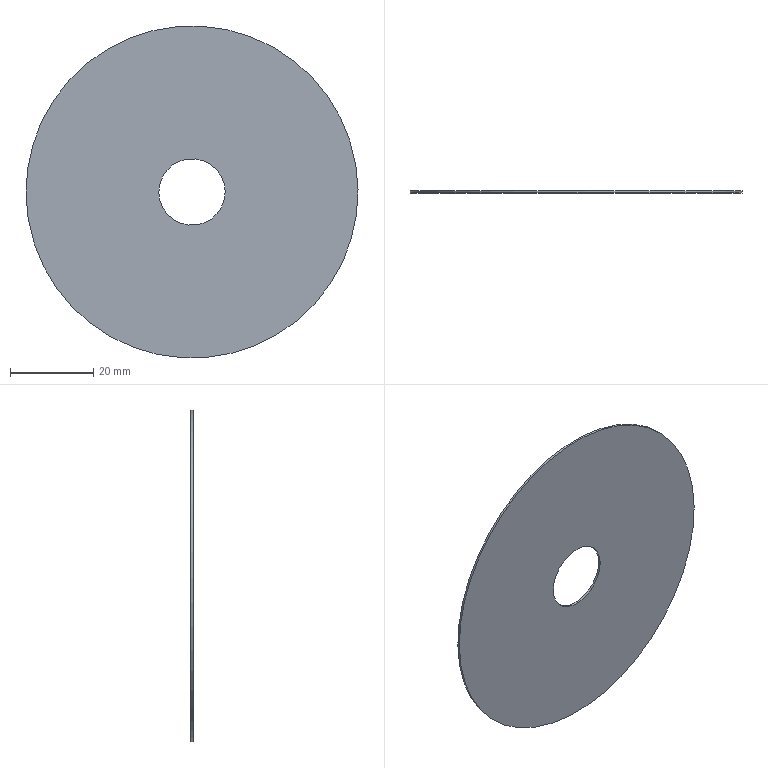Component | NX | BLADE | 1 solid | 4 faces | box 80 x 0.5 x 80 mm | volume 2413 mm3 | cylinder 2 | plane 2 | commonest cylinder face diameters 80 x1 16 x1
STEP:
#1=CARTESIAN_POINT('',(0.,0.,0.));
#2=DIRECTION('',(0.,0.,1.));
#3=DIRECTION('',(1.,0.,0.));
#4=AXIS2_PLACEMENT_3D('',#1,#2,#3);
#5=CARTESIAN_POINT('',(-471.672,8.4,378.045));
#6=VERTEX_POINT('',#5);
#7=CARTESIAN_POINT('',(-431.676,8.4,378.556));
#8=DIRECTION('',(0.,1.,0.));
#9=DIRECTION('',(-0.9999,0.,-0.01278));
#10=AXIS2_PLACEMENT_3D('',#7,#8,#9);
#11=CIRCLE('',#10,40.);
#12=CARTESIAN_POINT('',(-431.676,8.4,378.556));
#13=DIRECTION('',(0.,-1.,0.));
#14=DIRECTION('',(-0.01278,0.,0.9999));
#15=AXIS2_PLACEMENT_3D('',#12,#13,#14);
#16=CYLINDRICAL_SURFACE('',#15,40.);
#17=CARTESIAN_POINT('',(7.854,0.));
#18=DIRECTION('',(-1.,0.));
#19=VECTOR('',#18,1.);
#20=LINE('',#17,#19);
#21=(GEOMETRIC_REPRESENTATION_CONTEXT(2)PARAMETRIC_REPRESENTATION_CONTEXT()REPRESENTATION_CONTEXT('',''));
#22=DEFINITIONAL_REPRESENTATION('',(#20),#21);
#23=PCURVE('',#16,#22);
#24=CARTESIAN_POINT('',(-431.676,8.4,378.556));
#25=DIRECTION('',(0.,1.,0.));
#26=DIRECTION('',(0.01278,0.,-0.9999));
#27=AXIS2_PLACEMENT_3D('',#24,#25,#26);
#28=PLANE('',#27);
#29=CARTESIAN_POINT('',(0.,0.));
#30=DIRECTION('',(-0.,1.));
#31=AXIS2_PLACEMENT_2D('',#29,#30);
#32=CIRCLE('',#31,40.);
#33=(GEOMETRIC_REPRESENTATION_CONTEXT(2)PARAMETRIC_REPRESENTATION_CONTEXT()REPRESENTATION_CONTEXT('',''));
#34=DEFINITIONAL_REPRESENTATION('',(#32),#33);
#35=PCURVE('',#28,#34);
#36=SURFACE_CURVE('',#11,(#23,#35),.PCURVE_S1.);
#37=EDGE_CURVE('',#6,#6,#36,.T.);
#38=ORIENTED_EDGE('',*,*,#37,.F.);
#39=CARTESIAN_POINT('',(-471.672,7.9,378.045));
#40=VERTEX_POINT('',#39);
#41=CARTESIAN_POINT('',(-471.672,8.4,378.045));
#42=CARTESIAN_POINT('',(-471.672,7.9,378.045));
#43=B_SPLINE_CURVE_WITH_KNOTS('',1,(#41,#42),.UNSPECIFIED.,.F.,.F.,(2,2),(0.,0.5),.PIECEWISE_BEZIER_KNOTS.);
#44=CARTESIAN_POINT('',(7.854,0.));
#45=DIRECTION('',(0.,1.));
#46=VECTOR('',#45,1.);
#47=LINE('',#44,#46);
#48=(GEOMETRIC_REPRESENTATION_CONTEXT(2)PARAMETRIC_REPRESENTATION_CONTEXT()REPRESENTATION_CONTEXT('',''));
#49=DEFINITIONAL_REPRESENTATION('',(#47),#48);
#50=PCURVE('',#16,#49);
#51=CARTESIAN_POINT('',(1.571,0.));
#52=DIRECTION('',(0.,1.));
#53=VECTOR('',#52,1.);
#54=LINE('',#51,#53);
#55=(GEOMETRIC_REPRESENTATION_CONTEXT(2)PARAMETRIC_REPRESENTATION_CONTEXT()REPRESENTATION_CONTEXT('',''));
#56=DEFINITIONAL_REPRESENTATION('',(#54),#55);
#57=PCURVE('',#16,#56);
#58=SEAM_CURVE('',#43,(#50,#57),.PCURVE_S1.);
#59=EDGE_CURVE('',#6,#40,#58,.T.);
#60=ORIENTED_EDGE('',*,*,#59,.T.);
#61=CARTESIAN_POINT('',(-431.676,7.9,378.556));
#62=DIRECTION('',(0.,1.,0.));
#63=DIRECTION('',(-0.9999,0.,-0.01278));
#64=AXIS2_PLACEMENT_3D('',#61,#62,#63);
#65=CIRCLE('',#64,40.);
#66=CARTESIAN_POINT('',(7.854,0.5));
#67=DIRECTION('',(-1.,0.));
#68=VECTOR('',#67,1.);
#69=LINE('',#66,#68);
#70=(GEOMETRIC_REPRESENTATION_CONTEXT(2)PARAMETRIC_REPRESENTATION_CONTEXT()REPRESENTATION_CONTEXT('',''));
#71=DEFINITIONAL_REPRESENTATION('',(#69),#70);
#72=PCURVE('',#16,#71);
#73=CARTESIAN_POINT('',(-431.676,7.9,378.556));
#74=DIRECTION('',(0.,1.,0.));
#75=DIRECTION('',(0.01278,0.,-0.9999));
#76=AXIS2_PLACEMENT_3D('',#73,#74,#75);
#77=PLANE('',#76);
#78=CARTESIAN_POINT('',(0.,0.));
#79=DIRECTION('',(-0.,1.));
#80=AXIS2_PLACEMENT_2D('',#78,#79);
#81=CIRCLE('',#80,40.);
#82=(GEOMETRIC_REPRESENTATION_CONTEXT(2)PARAMETRIC_REPRESENTATION_CONTEXT()REPRESENTATION_CONTEXT('',''));
#83=DEFINITIONAL_REPRESENTATION('',(#81),#82);
#84=PCURVE('',#77,#83);
#85=SURFACE_CURVE('',#65,(#72,#84),.PCURVE_S1.);
#86=EDGE_CURVE('',#40,#40,#85,.T.);
#87=ORIENTED_EDGE('',*,*,#86,.T.);
#88=ORIENTED_EDGE('',*,*,#59,.F.);
#89=EDGE_LOOP('',(#38,#60,#87,#88));
#90=FACE_BOUND('',#89,.T.);
#91=ADVANCED_FACE('',(#90),#16,.T.);
#92=CARTESIAN_POINT('',(-439.675,8.4,378.454));
#93=VERTEX_POINT('',#92);
#94=CARTESIAN_POINT('',(-431.676,8.4,378.556));
#95=DIRECTION('',(0.,1.,0.));
#96=DIRECTION('',(-0.9999,0.,-0.01278));
#97=AXIS2_PLACEMENT_3D('',#94,#95,#96);
#98=CIRCLE('',#97,8.);
#99=CARTESIAN_POINT('',(-431.676,8.4,378.556));
#100=DIRECTION('',(0.,-1.,0.));
#101=DIRECTION('',(-0.01278,0.,0.9999));
#102=AXIS2_PLACEMENT_3D('',#99,#100,#101);
#103=CYLINDRICAL_SURFACE('',#102,8.);
#104=CARTESIAN_POINT('',(7.854,0.));
#105=DIRECTION('',(-1.,0.));
#106=VECTOR('',#105,1.);
#107=LINE('',#104,#106);
#108=(GEOMETRIC_REPRESENTATION_CONTEXT(2)PARAMETRIC_REPRESENTATION_CONTEXT()REPRESENTATION_CONTEXT('',''));
#109=DEFINITIONAL_REPRESENTATION('',(#107),#108);
#110=PCURVE('',#103,#109);
#111=CARTESIAN_POINT('',(0.,0.));
#112=DIRECTION('',(0.,1.));
#113=AXIS2_PLACEMENT_2D('',#111,#112);
#114=CIRCLE('',#113,8.);
#115=(GEOMETRIC_REPRESENTATION_CONTEXT(2)PARAMETRIC_REPRESENTATION_CONTEXT()REPRESENTATION_CONTEXT('',''));
#116=DEFINITIONAL_REPRESENTATION('',(#114),#115);
#117=PCURVE('',#28,#116);
#118=SURFACE_CURVE('',#98,(#110,#117),.PCURVE_S1.);
#119=EDGE_CURVE('',#93,#93,#118,.T.);
#120=ORIENTED_EDGE('',*,*,#119,.F.);
#121=CARTESIAN_POINT('',(-439.675,7.9,378.454));
#122=VERTEX_POINT('',#121);
#123=CARTESIAN_POINT('',(-439.675,8.4,378.454));
#124=CARTESIAN_POINT('',(-439.675,7.9,378.454));
#125=B_SPLINE_CURVE_WITH_KNOTS('',1,(#123,#124),.UNSPECIFIED.,.F.,.F.,(2,2),(0.,0.5),.PIECEWISE_BEZIER_KNOTS.);
#126=CARTESIAN_POINT('',(7.854,0.));
#127=DIRECTION('',(0.,1.));
#128=VECTOR('',#127,1.);
#129=LINE('',#126,#128);
#130=(GEOMETRIC_REPRESENTATION_CONTEXT(2)PARAMETRIC_REPRESENTATION_CONTEXT()REPRESENTATION_CONTEXT('',''));
#131=DEFINITIONAL_REPRESENTATION('',(#129),#130);
#132=PCURVE('',#103,#131);
#133=CARTESIAN_POINT('',(1.571,0.));
#134=DIRECTION('',(0.,1.));
#135=VECTOR('',#134,1.);
#136=LINE('',#133,#135);
#137=(GEOMETRIC_REPRESENTATION_CONTEXT(2)PARAMETRIC_REPRESENTATION_CONTEXT()REPRESENTATION_CONTEXT('',''));
#138=DEFINITIONAL_REPRESENTATION('',(#136),#137);
#139=PCURVE('',#103,#138);
#140=SEAM_CURVE('',#125,(#132,#139),.PCURVE_S1.);
#141=EDGE_CURVE('',#93,#122,#140,.T.);
#142=ORIENTED_EDGE('',*,*,#141,.T.);
#143=CARTESIAN_POINT('',(-431.676,7.9,378.556));
#144=DIRECTION('',(0.,1.,0.));
#145=DIRECTION('',(-0.9999,0.,-0.01278));
#146=AXIS2_PLACEMENT_3D('',#143,#144,#145);
#147=CIRCLE('',#146,8.);
#148=CARTESIAN_POINT('',(7.854,0.5));
#149=DIRECTION('',(-1.,0.));
#150=VECTOR('',#149,1.);
#151=LINE('',#148,#150);
#152=(GEOMETRIC_REPRESENTATION_CONTEXT(2)PARAMETRIC_REPRESENTATION_CONTEXT()REPRESENTATION_CONTEXT('',''));
#153=DEFINITIONAL_REPRESENTATION('',(#151),#152);
#154=PCURVE('',#103,#153);
#155=CARTESIAN_POINT('',(0.,0.));
#156=DIRECTION('',(0.,1.));
#157=AXIS2_PLACEMENT_2D('',#155,#156);
#158=CIRCLE('',#157,8.);
#159=(GEOMETRIC_REPRESENTATION_CONTEXT(2)PARAMETRIC_REPRESENTATION_CONTEXT()REPRESENTATION_CONTEXT('',''));
#160=DEFINITIONAL_REPRESENTATION('',(#158),#159);
#161=PCURVE('',#77,#160);
#162=SURFACE_CURVE('',#147,(#154,#161),.PCURVE_S1.);
#163=EDGE_CURVE('',#122,#122,#162,.T.);
#164=ORIENTED_EDGE('',*,*,#163,.T.);
#165=ORIENTED_EDGE('',*,*,#141,.F.);
#166=EDGE_LOOP('',(#120,#142,#164,#165));
#167=FACE_BOUND('',#166,.F.);
#168=ADVANCED_FACE('',(#167),#103,.F.);
#169=ORIENTED_EDGE('',*,*,#37,.T.);
#170=EDGE_LOOP('',(#169));
#171=FACE_BOUND('',#170,.T.);
#172=ORIENTED_EDGE('',*,*,#119,.F.);
#173=EDGE_LOOP('',(#172));
#174=FACE_BOUND('',#173,.T.);
#175=ADVANCED_FACE('',(#171,#174),#28,.T.);
#176=ORIENTED_EDGE('',*,*,#86,.F.);
#177=EDGE_LOOP('',(#176));
#178=FACE_BOUND('',#177,.T.);
#179=ORIENTED_EDGE('',*,*,#163,.T.);
#180=EDGE_LOOP('',(#179));
#181=FACE_BOUND('',#180,.T.);
#182=ADVANCED_FACE('',(#178,#181),#77,.F.);
#183=CLOSED_SHELL('',(#91,#168,#175,#182));
#184=MANIFOLD_SOLID_BREP('',#183);
#185=(LENGTH_UNIT()NAMED_UNIT(*)SI_UNIT(.MILLI.,.METRE.));
#186=UNCERTAINTY_MEASURE_WITH_UNIT(LENGTH_MEASURE(0.00001),#185,'','');
#187=(NAMED_UNIT(*)PLANE_ANGLE_UNIT()SI_UNIT($,.RADIAN.));
#188=(NAMED_UNIT(*)SI_UNIT($,.STERADIAN.)SOLID_ANGLE_UNIT());
#189=(GEOMETRIC_REPRESENTATION_CONTEXT(3)GLOBAL_UNCERTAINTY_ASSIGNED_CONTEXT((#186))GLOBAL_UNIT_ASSIGNED_CONTEXT((#185,#187,#188))REPRESENTATION_CONTEXT('',''));
#190=ADVANCED_BREP_SHAPE_REPRESENTATION('',(#4,#184),#189);